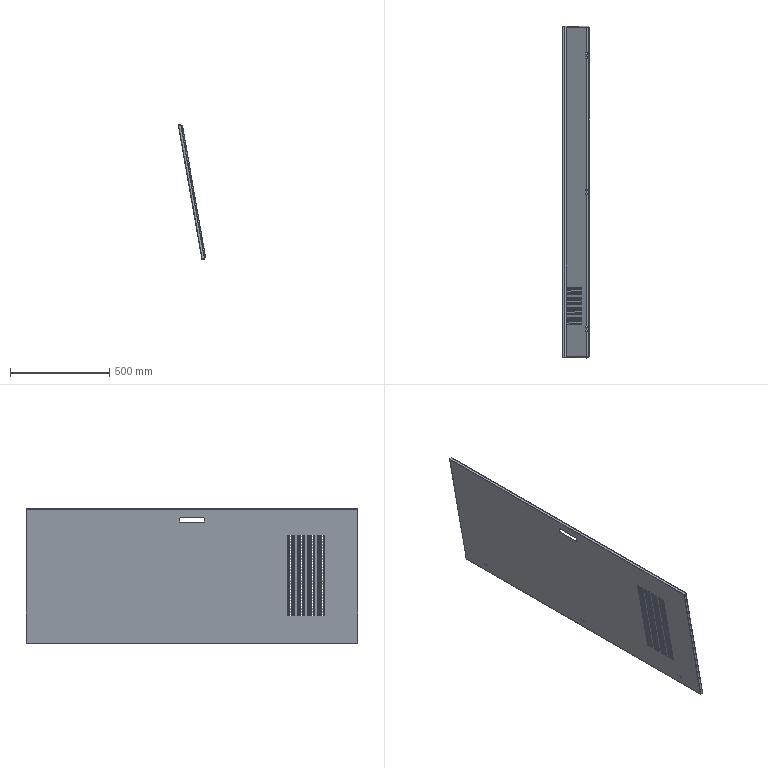Component | SolidWorks | KSHE-016.4-1_KSHE-016.017-1 | 1 solid | 924 faces | volume 1831885 mm3 | plane 888 | cylinder 28 | spline 8 | commonest cylinder face diameters 6 x16 3.2 x4 0.2 x4 3 x4